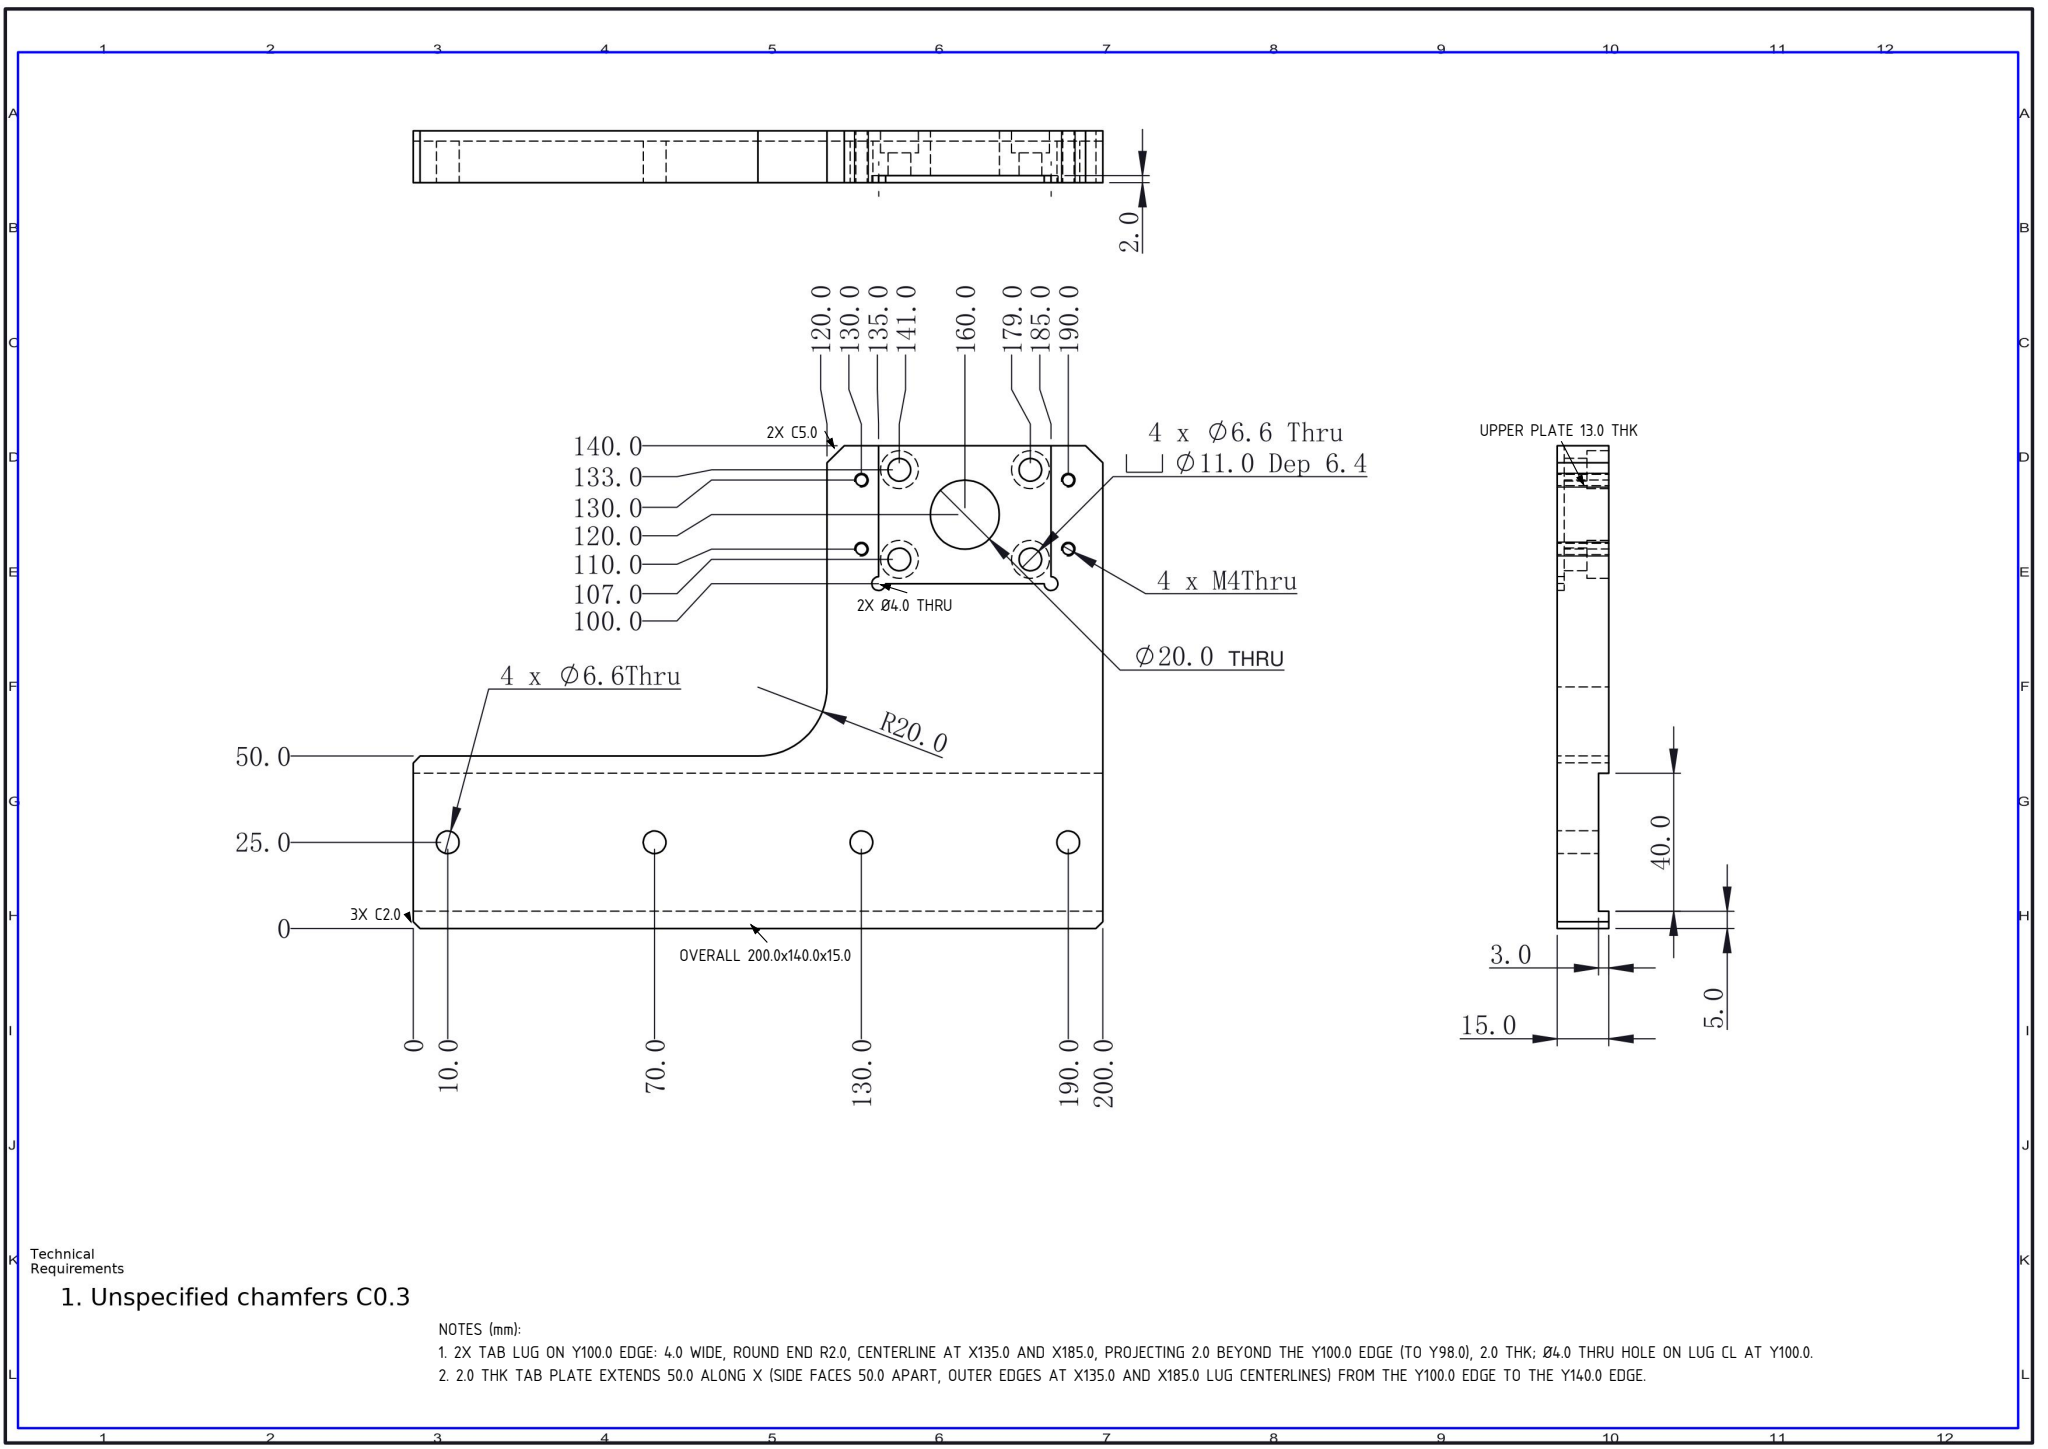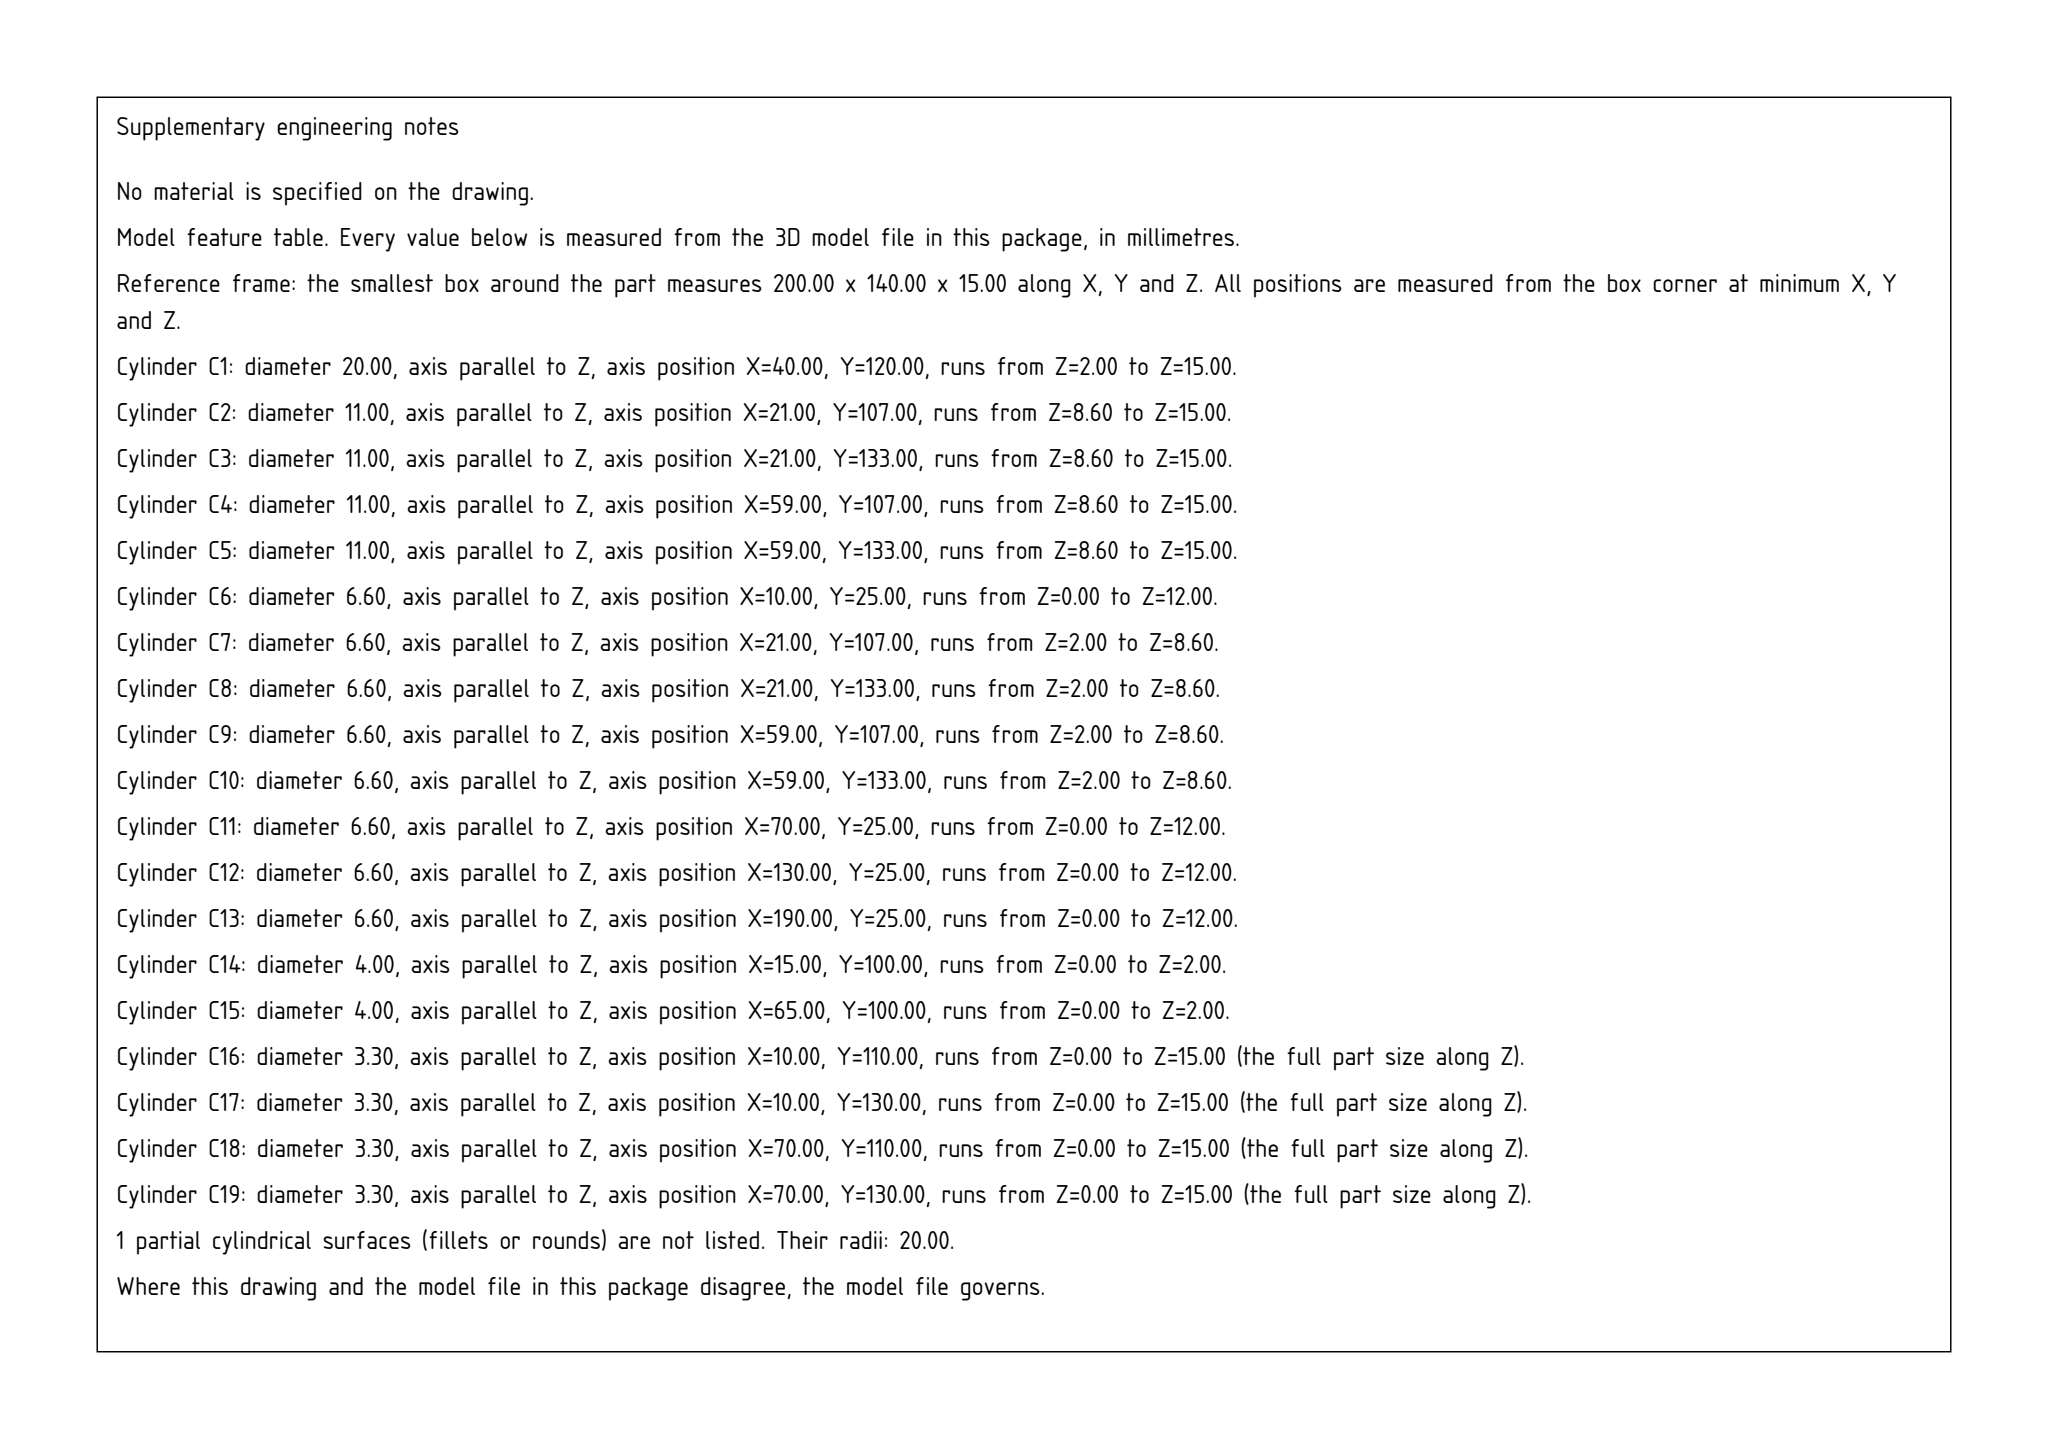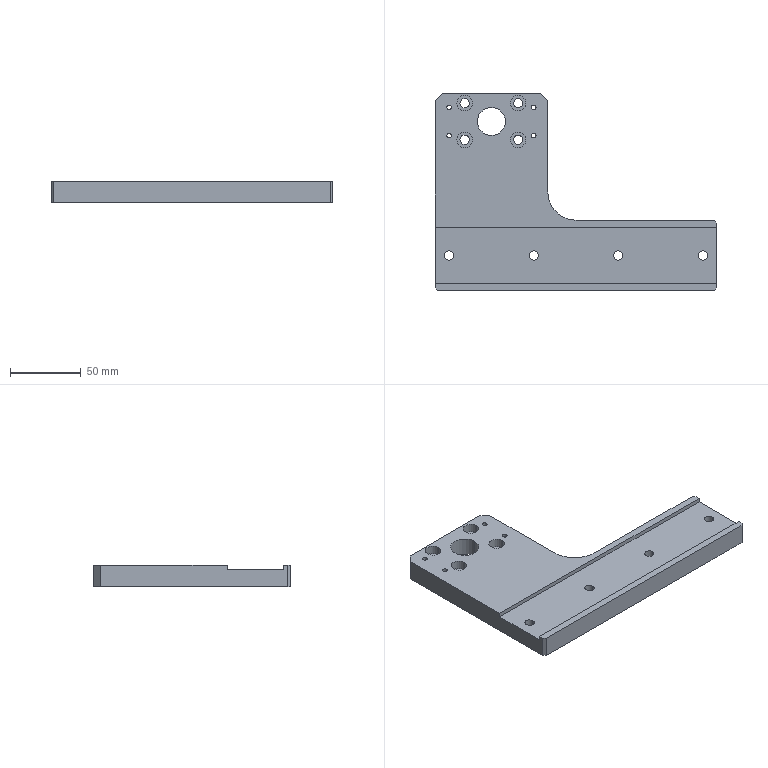Part | SolidWorks | mm | 1 solid | 63 faces | box 200 x 140 x 15 mm | volume 221209 mm3 | cylinder 38 | plane 25 | commonest cylinder face diameters 6.6 x16 3.3 x8 11 x8 4 x3 20 x2 40 x1
Drawing notes:
OVERALL 200.0 x 140.0 x 15.0 | from the solid: bbox_xyz [200.0, 140.0, 15.0]
UPPER PLATE 13.0 THK; BACK FACE 2.0 ABOVE BASE BACK FACE | from the solid: z-planes 0.0, 2.0, 15.0; Ø20 THRU cyl length 13.0 (z2 to z15)
2X Ø4.0 THRU 2.0 THK TAB, CL ON Y100.0 EDGE AT X135.0 & X185.0 | from the solid: Ø4.0 z-cyls len 2.0 at (15,100) & (65,100) = X185.0/X135.0 mirrored; y-plane 100.0; z-plane 2.0
2X 5.0 x 5.0 CHAMFER (45°) AT THE TWO TOP CORNERS OF THE UPPER ARM; CHAMFER STARTS 5.0 BELOW THE Y140.0 EDGE (AT Y135.0) AND 5.0 IN FROM EACH ARM SIDE EDGE, THROUGH FULL 15.0 THICKNESS. | from the solid: inclined_planes: angle_to_xyz_axes [45,45,90], bbox_from [0,135,0] size [5,5,15] and bbox_from [75,135,0] size [5,5,15]
3X 2.0 x 2.0 CHAMFER (45°) AT THE BASE OUTER CORNERS (BOTH CORNERS ON THE Y0 EDGE AND THE OUTBOARD CORNER ON THE Y50.0 EDGE), THROUGH FULL 15.0 THICKNESS. NOT COVERED BY GENERAL NOTE C0.3. | from the solid: inclined_planes: 45° faces bbox_from [0,0,0], [198,0,0], [198,48,0], each size [2,2,15]
2X TAB LUG ON Y100.0 EDGE: 4.0 WIDE, ROUND END R2.0, CENTERLINE AT X135.0 AND X185.0, PROJECTING 2.0 BEYOND THE Y100.0 EDGE (TO Y98.0), 2.0 THK; Ø4.0 THRU HOLE ON LUG CL AT Y100.0. | from the solid: concave arcs Ø4.0 z-axis at (15,100) and (65,100), z 0->2, 270°; plane z=2.0 extent x[13,67] y[98,140]; plane y=100 extent x[17,63] z[0,2]
2.0 THK TAB PLATE EXTENDS 50.0 ALONG X (SIDE FACES 50.0 APART, OUTER EDGES AT X135.0 AND X185.0 LUG CENTERLINES) FROM THE Y100.0 EDGE TO THE Y140.0 EDGE. | from the solid: planes x=15.0 and x=65.0, extent y[102,140] z[0,2]; plane z=2.0 extent x[13,67] y[98,140]
build123d program:
from build123d import *

# Parameters (mm, degrees)
BOSS_EXTRUDE1_DEPTH                             = 15
SKETCH2_W                                       = 200
SKETCH2_H                                       = 40
CUT_EXTRUDE1_DEPTH                              = 3
CUT_EXTRUDE2_DEPTH                              = 245.591
CUT_EXTRUDE2_DEPTH_BACK                         = 245.591
SKETCH3_R                                       = 10
M6_HEX_SOCKET_HEAD_CAP_SCREW_CBORE1_D           = 6.6
M6_HEX_SOCKET_HEAD_CAP_SCREW_CBORE1_CBORE_D     = 11
M6_HEX_SOCKET_HEAD_CAP_SCREW_CBORE1_CBORE_DEPTH = 6.4
M4_TAPPED_HOLE1_D                               = 3.3
M6_CLEARANCE_HOLE1_D                            = 6.6
FILLET1_R                                       = 20
CHAMFER1_SIZE                                   = 5
CHAMFER2_SIZE                                   = 2
SKETCH10_W                                      = 50
SKETCH10_H                                      = 40
CUT_EXTRUDE3_DEPTH                              = 2
SKETCH11_R                                      = 2
CUT_EXTRUDE4_DEPTH                              = 2


with BuildPart() as part:
    # Sketch1 → Boss-Extrude1 (new body)
    with BuildSketch(Plane.XY):
        Polygon((0, 50), (0, 0), (-200, 0), (-200, 140), (-120, 140), (-120, 50), align=None)
    extrude(amount=BOSS_EXTRUDE1_DEPTH)

    # Sketch2 → Cut-Extrude1 (cut)
    with BuildSketch(Plane(origin=(0, 0, 15), x_dir=(-1, 0, 0), z_dir=(0, 0, -1))):
        with Locations((100, 25)):
            Rectangle(SKETCH2_W, SKETCH2_H)
    extrude(amount=CUT_EXTRUDE1_DEPTH, mode=Mode.SUBTRACT)

    # Sketch3 → Cut-Extrude2 (cut, two sides: drawn at the far end of the back side and taken through both)
    with BuildSketch(Plane.XY.offset(15).offset(-CUT_EXTRUDE2_DEPTH_BACK)):
        with Locations((-160, 120)):
            Circle(SKETCH3_R)
    extrude(amount=CUT_EXTRUDE2_DEPTH + CUT_EXTRUDE2_DEPTH_BACK, mode=Mode.SUBTRACT)

    # M6 Hex Socket Head Cap Screw CBORE1 (through all)
    with Locations(Plane.XY.offset(15)):
        with Locations((-179, 133), (-141, 133), (-179, 107), (-141, 107)):
            CounterBoreHole(M6_HEX_SOCKET_HEAD_CAP_SCREW_CBORE1_D / 2, M6_HEX_SOCKET_HEAD_CAP_SCREW_CBORE1_CBORE_D / 2, M6_HEX_SOCKET_HEAD_CAP_SCREW_CBORE1_CBORE_DEPTH)

    # M4 Tapped Hole1 (through all)
    with Locations(Plane.XY.offset(15)):
        with Locations((-190, 110), (-190, 130), (-130, 110), (-130, 130)):
            Hole(M4_TAPPED_HOLE1_D / 2)

    # M6 Clearance Hole1 (through all)
    with Locations(Plane.XY.offset(12)):
        with Locations((-190, 25), (-130, 25), (-70, 25), (-10, 25)):
            Hole(M6_CLEARANCE_HOLE1_D / 2)

    # Fillet1
    fillet1_edges = [part.edges().sort_by_distance(p)[0] for p in [
        (-120, 50, 7.5),
    ]]
    fillet(fillet1_edges, radius=FILLET1_R)

    # Chamfer1
    chamfer1_edges = [part.edges().sort_by_distance(p)[0] for p in [
        (-200, 140, 7.5),
        (-120, 140, 7.5),
    ]]
    chamfer(chamfer1_edges, length=CHAMFER1_SIZE)

    # Chamfer2
    chamfer2_edges = [part.edges().sort_by_distance(p)[0] for p in [
        (-200, 0, 7.5),
        (0, 50, 7.5),
        (0, 0, 7.5),
    ]]
    chamfer(chamfer2_edges, length=CHAMFER2_SIZE)

    # Sketch10 → Cut-Extrude3 (cut)
    with BuildSketch(Plane(origin=(0, 0, 0), x_dir=(-1, 0, 0), z_dir=(0, 0, -1))):
        with Locations((160, 120)):
            Rectangle(SKETCH10_W, SKETCH10_H)
    extrude(amount=-CUT_EXTRUDE3_DEPTH, mode=Mode.SUBTRACT)

    # Sketch11 → Cut-Extrude4 (cut)
    with BuildSketch(Plane(origin=(0, 0, 0), x_dir=(-1, 0, 0), z_dir=(0, 0, -1))):
        with Locations((135, 100)):
            Circle(SKETCH11_R)
        with Locations((185, 100)):
            Circle(SKETCH11_R)
    extrude(amount=-CUT_EXTRUDE4_DEPTH, mode=Mode.SUBTRACT)


solid = part.part